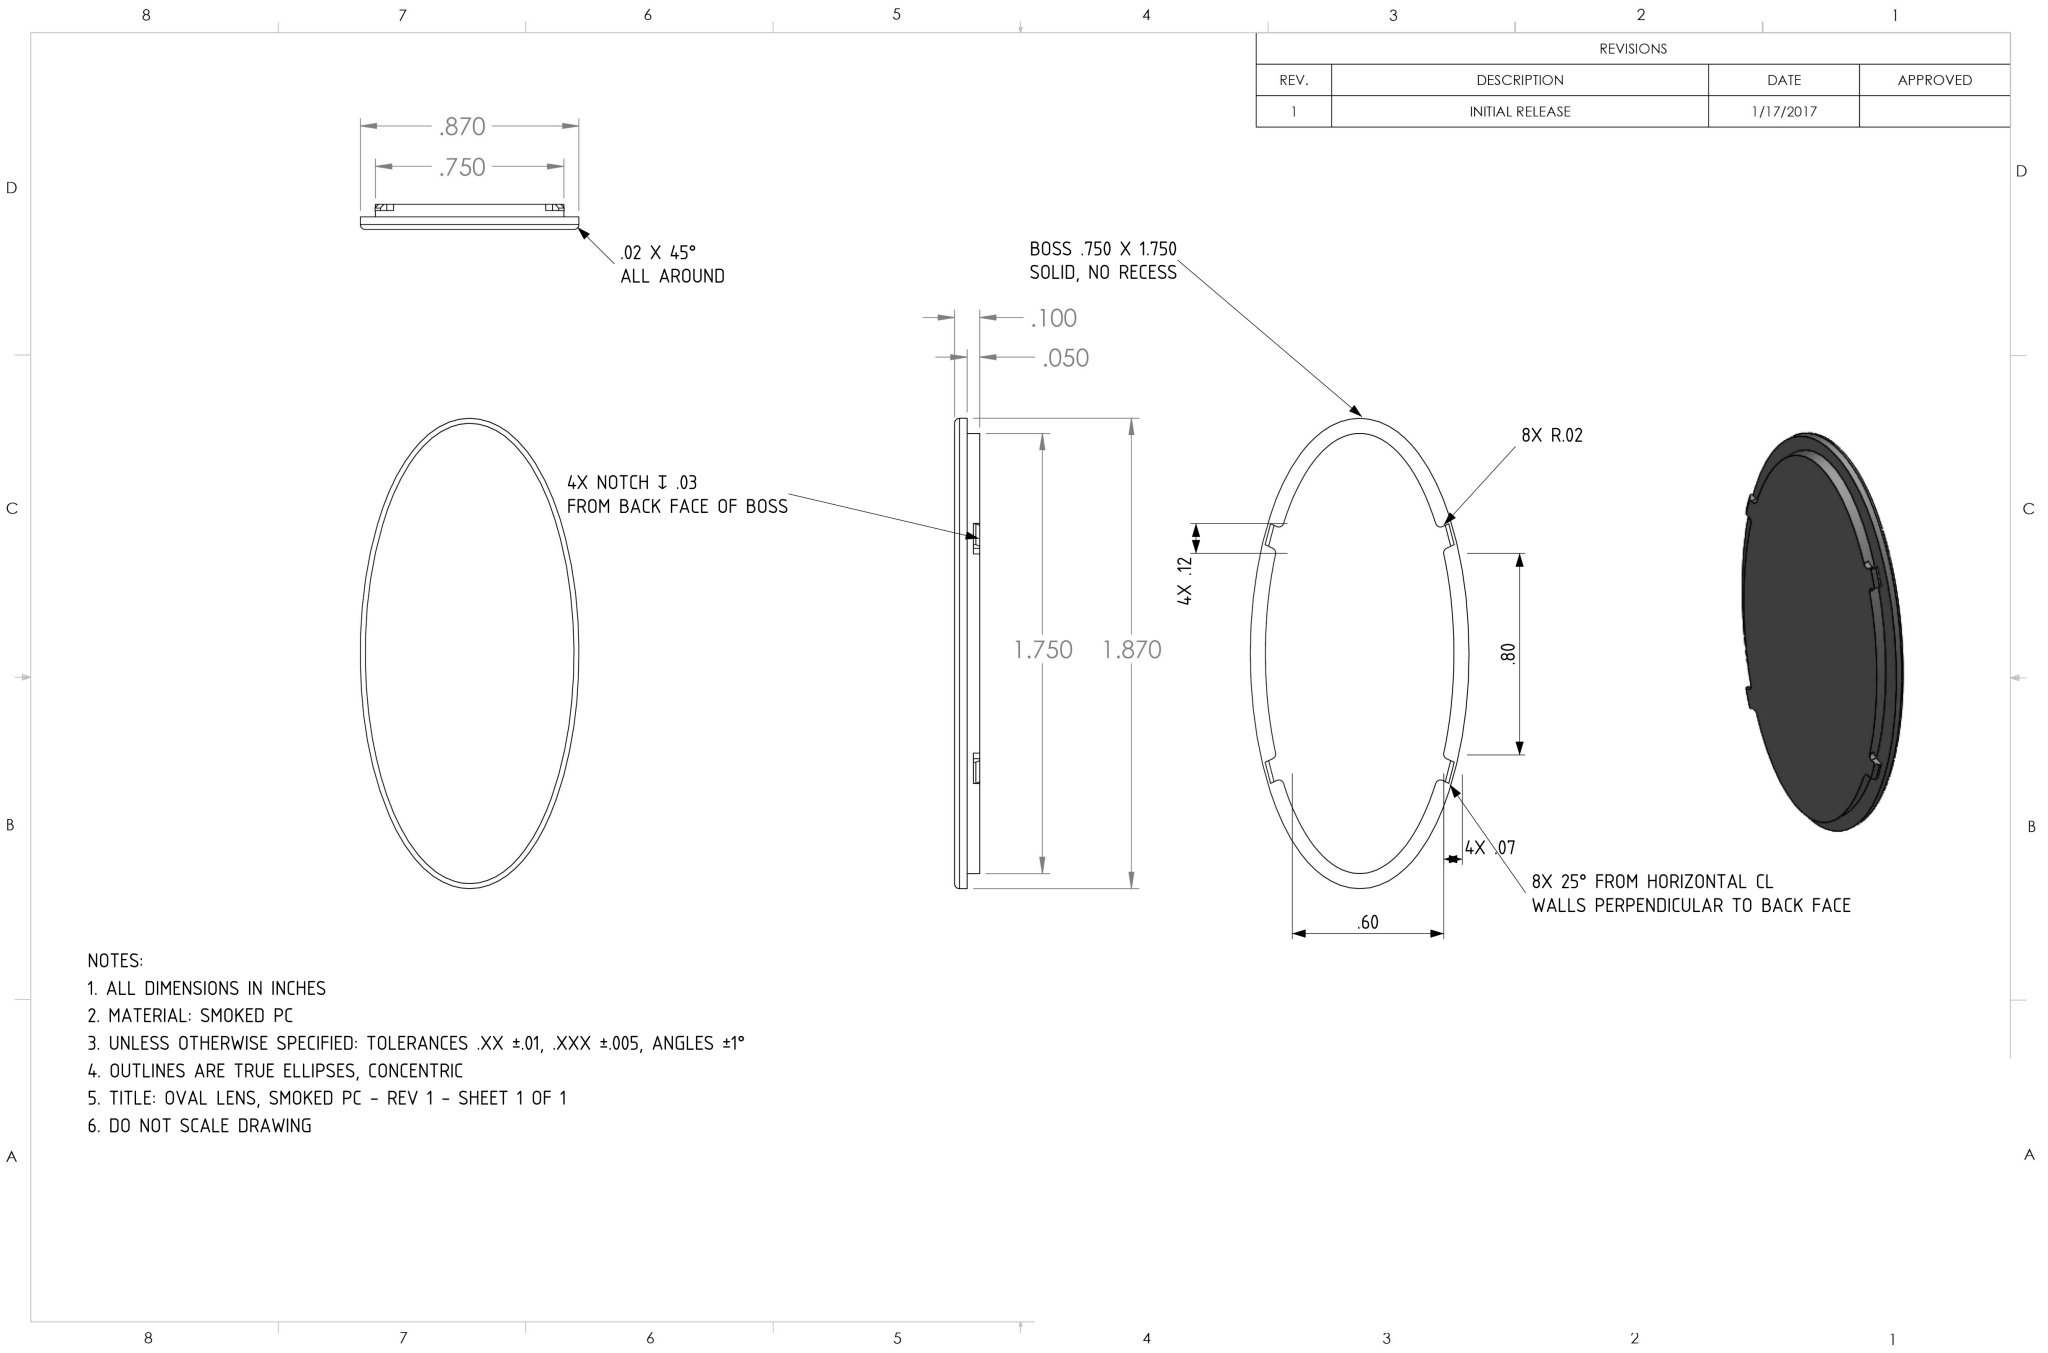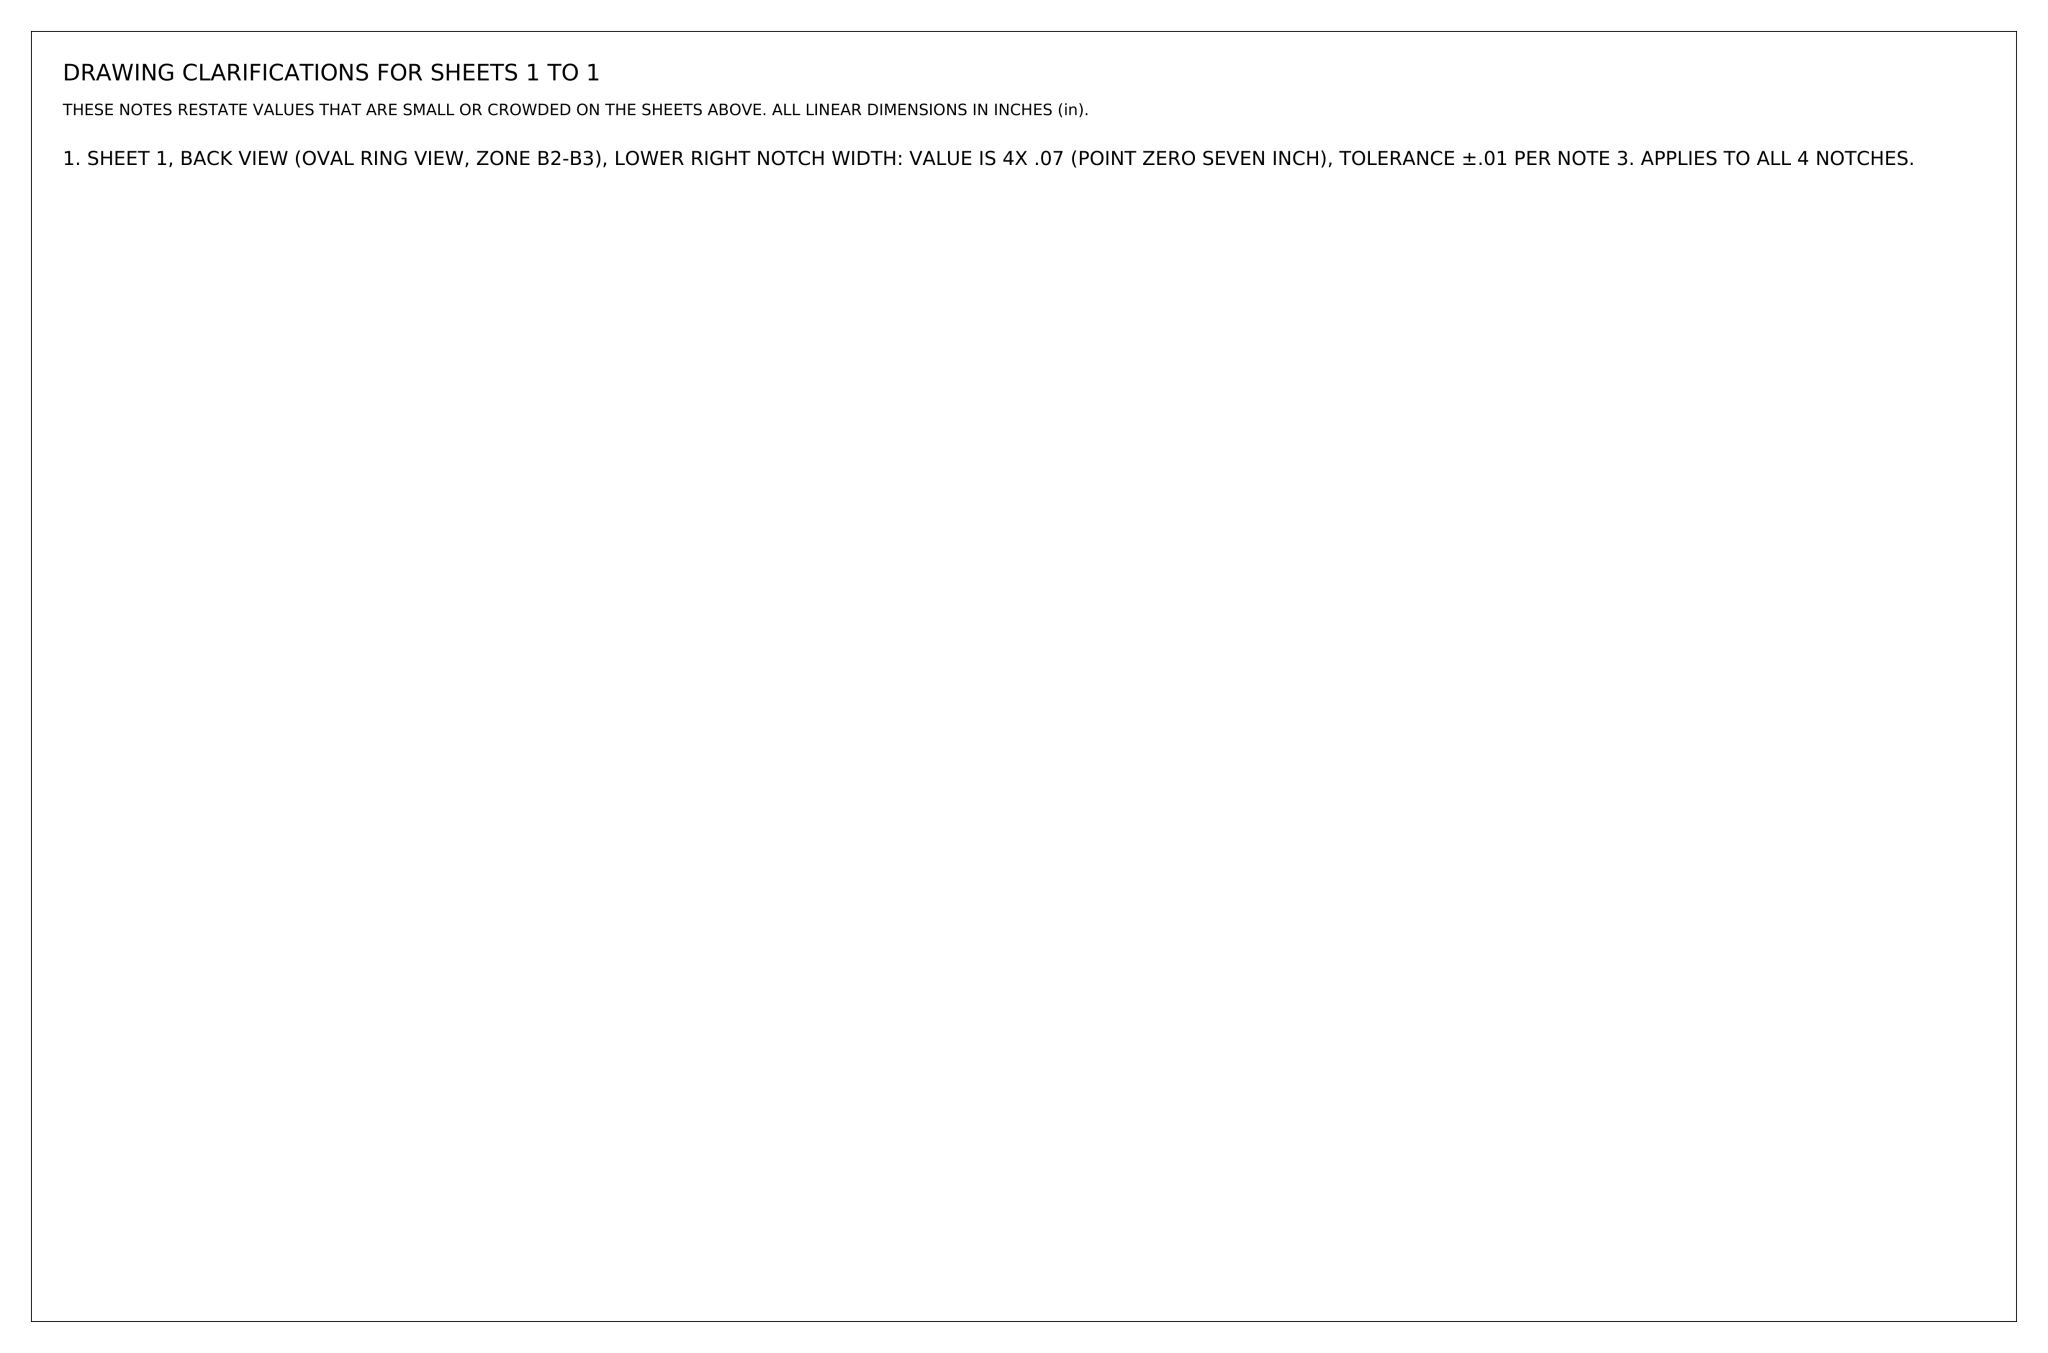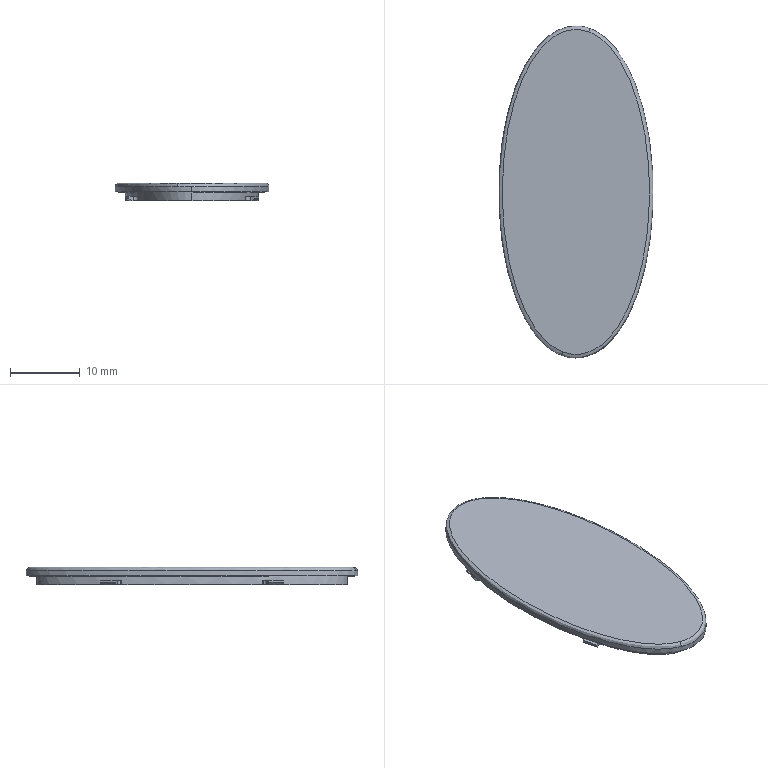Part | NX | drawing in inches | 1 solid | 39 faces | box 22.1 x 47.5 x 2.54 mm | volume 1899 mm3 | plane 15 | spline 14 | cylinder 10 | commonest cylinder face diameters 1.016 x10